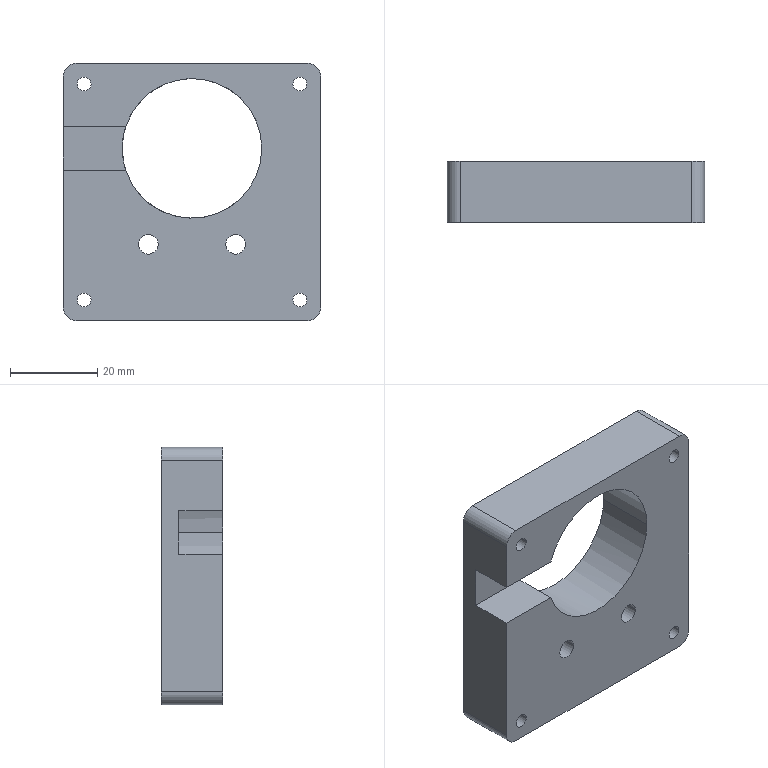Component | SolidWorks | MotorPlate-1 | 1 solid | 33 faces | box 59 x 14 x 59 mm | volume 34785 mm3 | cylinder 22 | plane 11 | commonest cylinder face diameters 3.2 x8 8 x4 4.5 x4 6 x4 32 x2 | material 6061 Alloy
STEP:
#1=CARTESIAN_POINT('',(-2.148,0.2347,12.047));
#2=VERTEX_POINT('',#1);
#3=CARTESIAN_POINT('',(-2.462,0.2347,12.047));
#4=VERTEX_POINT('',#3);
#5=CARTESIAN_POINT('',(-2.305,0.2347,12.047));
#6=DIRECTION('',(-0.,1.,-0.));
#7=DIRECTION('',(-1.,-0.,0.));
#8=AXIS2_PLACEMENT_3D('',#5,#6,#7);
#9=CIRCLE('',#8,0.1575);
#10=EDGE_CURVE('',#2,#4,#9,.T.);
#11=ORIENTED_EDGE('',*,*,#10,.F.);
#12=CARTESIAN_POINT('',(-2.148,0.4118,12.047));
#13=VERTEX_POINT('',#12);
#14=CARTESIAN_POINT('',(-2.148,0.2347,12.047));
#15=DIRECTION('',(-0.,1.,-0.));
#16=VECTOR('',#15,39.37);
#17=LINE('',#14,#16);
#18=EDGE_CURVE('',#2,#13,#17,.T.);
#19=ORIENTED_EDGE('',*,*,#18,.T.);
#20=CARTESIAN_POINT('',(-2.462,0.4118,12.047));
#21=VERTEX_POINT('',#20);
#22=CARTESIAN_POINT('',(-2.305,0.4118,12.047));
#23=DIRECTION('',(-0.,1.,-0.));
#24=DIRECTION('',(-1.,-0.,0.));
#25=AXIS2_PLACEMENT_3D('',#22,#23,#24);
#26=CIRCLE('',#25,0.1575);
#27=EDGE_CURVE('',#13,#21,#26,.T.);
#28=ORIENTED_EDGE('',*,*,#27,.T.);
#29=CARTESIAN_POINT('',(-2.462,0.2347,12.047));
#30=DIRECTION('',(-0.,1.,-0.));
#31=VECTOR('',#30,39.37);
#32=LINE('',#29,#31);
#33=EDGE_CURVE('',#4,#21,#32,.T.);
#34=ORIENTED_EDGE('',*,*,#33,.F.);
#35=EDGE_LOOP('',(#11,#19,#28,#34));
#36=FACE_OUTER_BOUND('',#35,.T.);
#37=CARTESIAN_POINT('',(-2.305,0.2347,12.047));
#38=DIRECTION('',(-0.,1.,-0.));
#39=DIRECTION('',(-1.,-0.,0.));
#40=AXIS2_PLACEMENT_3D('',#37,#38,#39);
#41=CYLINDRICAL_SURFACE('',#40,0.1575);
#42=ADVANCED_FACE('',(#36),#41,.F.);
#43=CARTESIAN_POINT('',(-1.36,0.2347,12.047));
#44=VERTEX_POINT('',#43);
#45=CARTESIAN_POINT('',(-1.675,0.2347,12.047));
#46=VERTEX_POINT('',#45);
#47=CARTESIAN_POINT('',(-1.518,0.2347,12.047));
#48=DIRECTION('',(-0.,1.,-0.));
#49=DIRECTION('',(-1.,-0.,0.));
#50=AXIS2_PLACEMENT_3D('',#47,#48,#49);
#51=CIRCLE('',#50,0.1575);
#52=EDGE_CURVE('',#44,#46,#51,.T.);
#53=ORIENTED_EDGE('',*,*,#52,.F.);
#54=CARTESIAN_POINT('',(-1.36,0.4118,12.047));
#55=VERTEX_POINT('',#54);
#56=CARTESIAN_POINT('',(-1.36,0.2347,12.047));
#57=DIRECTION('',(-0.,1.,-0.));
#58=VECTOR('',#57,39.37);
#59=LINE('',#56,#58);
#60=EDGE_CURVE('',#44,#55,#59,.T.);
#61=ORIENTED_EDGE('',*,*,#60,.T.);
#62=CARTESIAN_POINT('',(-1.675,0.4118,12.047));
#63=VERTEX_POINT('',#62);
#64=CARTESIAN_POINT('',(-1.518,0.4118,12.047));
#65=DIRECTION('',(-0.,1.,-0.));
#66=DIRECTION('',(-1.,-0.,0.));
#67=AXIS2_PLACEMENT_3D('',#64,#65,#66);
#68=CIRCLE('',#67,0.1575);
#69=EDGE_CURVE('',#55,#63,#68,.T.);
#70=ORIENTED_EDGE('',*,*,#69,.T.);
#71=CARTESIAN_POINT('',(-1.675,0.2347,12.047));
#72=DIRECTION('',(-0.,1.,-0.));
#73=VECTOR('',#72,39.37);
#74=LINE('',#71,#73);
#75=EDGE_CURVE('',#46,#63,#74,.T.);
#76=ORIENTED_EDGE('',*,*,#75,.F.);
#77=EDGE_LOOP('',(#53,#61,#70,#76));
#78=FACE_OUTER_BOUND('',#77,.T.);
#79=CARTESIAN_POINT('',(-1.518,0.2347,12.047));
#80=DIRECTION('',(-0.,1.,-0.));
#81=DIRECTION('',(-1.,-0.,0.));
#82=AXIS2_PLACEMENT_3D('',#79,#80,#81);
#83=CYLINDRICAL_SURFACE('',#82,0.1575);
#84=ADVANCED_FACE('',(#78),#83,.F.);
#85=CARTESIAN_POINT('',(-0.8739,0.4118,11.545));
#86=VERTEX_POINT('',#85);
#87=CARTESIAN_POINT('',(-0.9999,0.4118,11.545));
#88=VERTEX_POINT('',#87);
#89=CARTESIAN_POINT('',(-0.9369,0.4118,11.545));
#90=DIRECTION('',(-0.,1.,-0.));
#91=DIRECTION('',(-1.,0.,0.));
#92=AXIS2_PLACEMENT_3D('',#89,#90,#91);
#93=CIRCLE('',#92,0.06299);
#94=EDGE_CURVE('',#86,#88,#93,.T.);
#95=ORIENTED_EDGE('',*,*,#94,.T.);
#96=CARTESIAN_POINT('',(-0.9999,-0.1394,11.545));
#97=VERTEX_POINT('',#96);
#98=CARTESIAN_POINT('',(-0.9999,0.4118,11.545));
#99=DIRECTION('',(0.,-1.,0.));
#100=VECTOR('',#99,39.37);
#101=LINE('',#98,#100);
#102=EDGE_CURVE('',#88,#97,#101,.T.);
#103=ORIENTED_EDGE('',*,*,#102,.T.);
#104=CARTESIAN_POINT('',(-0.8739,-0.1394,11.545));
#105=VERTEX_POINT('',#104);
#106=CARTESIAN_POINT('',(-0.9369,-0.1394,11.545));
#107=DIRECTION('',(-0.,1.,-0.));
#108=DIRECTION('',(-1.,-0.,0.));
#109=AXIS2_PLACEMENT_3D('',#106,#107,#108);
#110=CIRCLE('',#109,0.06299);
#111=EDGE_CURVE('',#105,#97,#110,.T.);
#112=ORIENTED_EDGE('',*,*,#111,.F.);
#113=CARTESIAN_POINT('',(-0.8739,0.4118,11.545));
#114=DIRECTION('',(0.,-1.,0.));
#115=VECTOR('',#114,39.37);
#116=LINE('',#113,#115);
#117=EDGE_CURVE('',#86,#105,#116,.T.);
#118=ORIENTED_EDGE('',*,*,#117,.F.);
#119=EDGE_LOOP('',(#95,#103,#112,#118));
#120=FACE_OUTER_BOUND('',#119,.T.);
#121=CARTESIAN_POINT('',(-0.9369,0.4118,11.545));
#122=DIRECTION('',(0.,-1.,0.));
#123=DIRECTION('',(1.,0.,0.));
#124=AXIS2_PLACEMENT_3D('',#121,#122,#123);
#125=CYLINDRICAL_SURFACE('',#124,0.06299);
#126=ADVANCED_FACE('',(#120),#125,.F.);
#127=CARTESIAN_POINT('',(-2.823,0.4118,11.545));
#128=VERTEX_POINT('',#127);
#129=CARTESIAN_POINT('',(-2.949,0.4118,11.545));
#130=VERTEX_POINT('',#129);
#131=CARTESIAN_POINT('',(-2.886,0.4118,11.545));
#132=DIRECTION('',(-0.,1.,-0.));
#133=DIRECTION('',(-1.,0.,0.));
#134=AXIS2_PLACEMENT_3D('',#131,#132,#133);
#135=CIRCLE('',#134,0.06299);
#136=EDGE_CURVE('',#128,#130,#135,.T.);
#137=ORIENTED_EDGE('',*,*,#136,.T.);
#138=CARTESIAN_POINT('',(-2.949,-0.1394,11.545));
#139=VERTEX_POINT('',#138);
#140=CARTESIAN_POINT('',(-2.949,0.4118,11.545));
#141=DIRECTION('',(0.,-1.,0.));
#142=VECTOR('',#141,39.37);
#143=LINE('',#140,#142);
#144=EDGE_CURVE('',#130,#139,#143,.T.);
#145=ORIENTED_EDGE('',*,*,#144,.T.);
#146=CARTESIAN_POINT('',(-2.823,-0.1394,11.545));
#147=VERTEX_POINT('',#146);
#148=CARTESIAN_POINT('',(-2.886,-0.1394,11.545));
#149=DIRECTION('',(-0.,1.,-0.));
#150=DIRECTION('',(-1.,-0.,0.));
#151=AXIS2_PLACEMENT_3D('',#148,#149,#150);
#152=CIRCLE('',#151,0.06299);
#153=EDGE_CURVE('',#147,#139,#152,.T.);
#154=ORIENTED_EDGE('',*,*,#153,.F.);
#155=CARTESIAN_POINT('',(-2.823,0.4118,11.545));
#156=DIRECTION('',(0.,-1.,0.));
#157=VECTOR('',#156,39.37);
#158=LINE('',#155,#157);
#159=EDGE_CURVE('',#128,#147,#158,.T.);
#160=ORIENTED_EDGE('',*,*,#159,.F.);
#161=EDGE_LOOP('',(#137,#145,#154,#160));
#162=FACE_OUTER_BOUND('',#161,.T.);
#163=CARTESIAN_POINT('',(-2.886,0.4118,11.545));
#164=DIRECTION('',(0.,-1.,0.));
#165=DIRECTION('',(1.,0.,0.));
#166=AXIS2_PLACEMENT_3D('',#163,#164,#165);
#167=CYLINDRICAL_SURFACE('',#166,0.06299);
#168=ADVANCED_FACE('',(#162),#167,.F.);
#169=CARTESIAN_POINT('',(-2.823,0.4118,13.494));
#170=VERTEX_POINT('',#169);
#171=CARTESIAN_POINT('',(-2.949,0.4118,13.494));
#172=VERTEX_POINT('',#171);
#173=CARTESIAN_POINT('',(-2.886,0.4118,13.494));
#174=DIRECTION('',(-0.,1.,-0.));
#175=DIRECTION('',(-1.,0.,0.));
#176=AXIS2_PLACEMENT_3D('',#173,#174,#175);
#177=CIRCLE('',#176,0.06299);
#178=EDGE_CURVE('',#170,#172,#177,.T.);
#179=ORIENTED_EDGE('',*,*,#178,.T.);
#180=CARTESIAN_POINT('',(-2.949,-0.1394,13.494));
#181=VERTEX_POINT('',#180);
#182=CARTESIAN_POINT('',(-2.949,0.4118,13.494));
#183=DIRECTION('',(0.,-1.,0.));
#184=VECTOR('',#183,39.37);
#185=LINE('',#182,#184);
#186=EDGE_CURVE('',#172,#181,#185,.T.);
#187=ORIENTED_EDGE('',*,*,#186,.T.);
#188=CARTESIAN_POINT('',(-2.823,-0.1394,13.494));
#189=VERTEX_POINT('',#188);
#190=CARTESIAN_POINT('',(-2.886,-0.1394,13.494));
#191=DIRECTION('',(-0.,1.,-0.));
#192=DIRECTION('',(-1.,-0.,0.));
#193=AXIS2_PLACEMENT_3D('',#190,#191,#192);
#194=CIRCLE('',#193,0.06299);
#195=EDGE_CURVE('',#189,#181,#194,.T.);
#196=ORIENTED_EDGE('',*,*,#195,.F.);
#197=CARTESIAN_POINT('',(-2.823,0.4118,13.494));
#198=DIRECTION('',(0.,-1.,0.));
#199=VECTOR('',#198,39.37);
#200=LINE('',#197,#199);
#201=EDGE_CURVE('',#170,#189,#200,.T.);
#202=ORIENTED_EDGE('',*,*,#201,.F.);
#203=EDGE_LOOP('',(#179,#187,#196,#202));
#204=FACE_OUTER_BOUND('',#203,.T.);
#205=CARTESIAN_POINT('',(-2.886,0.4118,13.494));
#206=DIRECTION('',(0.,-1.,0.));
#207=DIRECTION('',(1.,0.,0.));
#208=AXIS2_PLACEMENT_3D('',#205,#206,#207);
#209=CYLINDRICAL_SURFACE('',#208,0.06299);
#210=ADVANCED_FACE('',(#204),#209,.F.);
#211=CARTESIAN_POINT('',(-0.8739,0.4118,13.494));
#212=VERTEX_POINT('',#211);
#213=CARTESIAN_POINT('',(-0.9999,0.4118,13.494));
#214=VERTEX_POINT('',#213);
#215=CARTESIAN_POINT('',(-0.9369,0.4118,13.494));
#216=DIRECTION('',(-0.,1.,-0.));
#217=DIRECTION('',(-1.,0.,0.));
#218=AXIS2_PLACEMENT_3D('',#215,#216,#217);
#219=CIRCLE('',#218,0.06299);
#220=EDGE_CURVE('',#212,#214,#219,.T.);
#221=ORIENTED_EDGE('',*,*,#220,.T.);
#222=CARTESIAN_POINT('',(-0.9999,-0.1394,13.494));
#223=VERTEX_POINT('',#222);
#224=CARTESIAN_POINT('',(-0.9999,0.4118,13.494));
#225=DIRECTION('',(0.,-1.,0.));
#226=VECTOR('',#225,39.37);
#227=LINE('',#224,#226);
#228=EDGE_CURVE('',#214,#223,#227,.T.);
#229=ORIENTED_EDGE('',*,*,#228,.T.);
#230=CARTESIAN_POINT('',(-0.8739,-0.1394,13.494));
#231=VERTEX_POINT('',#230);
#232=CARTESIAN_POINT('',(-0.9369,-0.1394,13.494));
#233=DIRECTION('',(-0.,1.,-0.));
#234=DIRECTION('',(-1.,-0.,0.));
#235=AXIS2_PLACEMENT_3D('',#232,#233,#234);
#236=CIRCLE('',#235,0.06299);
#237=EDGE_CURVE('',#231,#223,#236,.T.);
#238=ORIENTED_EDGE('',*,*,#237,.F.);
#239=CARTESIAN_POINT('',(-0.8739,0.4118,13.494));
#240=DIRECTION('',(0.,-1.,0.));
#241=VECTOR('',#240,39.37);
#242=LINE('',#239,#241);
#243=EDGE_CURVE('',#212,#231,#242,.T.);
#244=ORIENTED_EDGE('',*,*,#243,.F.);
#245=EDGE_LOOP('',(#221,#229,#238,#244));
#246=FACE_OUTER_BOUND('',#245,.T.);
#247=CARTESIAN_POINT('',(-0.9369,0.4118,13.494));
#248=DIRECTION('',(0.,-1.,0.));
#249=DIRECTION('',(1.,0.,0.));
#250=AXIS2_PLACEMENT_3D('',#247,#248,#249);
#251=CYLINDRICAL_SURFACE('',#250,0.06299);
#252=ADVANCED_FACE('',(#246),#251,.F.);
#253=CARTESIAN_POINT('',(-1.429,0.2347,12.047));
#254=VERTEX_POINT('',#253);
#255=CARTESIAN_POINT('',(-1.606,0.2347,12.047));
#256=VERTEX_POINT('',#255);
#257=CARTESIAN_POINT('',(-1.518,0.2347,12.047));
#258=DIRECTION('',(-0.,1.,-0.));
#259=DIRECTION('',(-1.,-0.,0.));
#260=AXIS2_PLACEMENT_3D('',#257,#258,#259);
#261=CIRCLE('',#260,0.08858);
#262=EDGE_CURVE('',#254,#256,#261,.T.);
#263=ORIENTED_EDGE('',*,*,#262,.T.);
#264=CARTESIAN_POINT('',(-1.606,-0.1394,12.047));
#265=VERTEX_POINT('',#264);
#266=CARTESIAN_POINT('',(-1.606,0.4118,12.047));
#267=DIRECTION('',(0.,-1.,0.));
#268=VECTOR('',#267,39.37);
#269=LINE('',#266,#268);
#270=EDGE_CURVE('',#256,#265,#269,.T.);
#271=ORIENTED_EDGE('',*,*,#270,.T.);
#272=CARTESIAN_POINT('',(-1.429,-0.1394,12.047));
#273=VERTEX_POINT('',#272);
#274=CARTESIAN_POINT('',(-1.518,-0.1394,12.047));
#275=DIRECTION('',(-0.,1.,-0.));
#276=DIRECTION('',(-1.,-0.,0.));
#277=AXIS2_PLACEMENT_3D('',#274,#275,#276);
#278=CIRCLE('',#277,0.08858);
#279=EDGE_CURVE('',#273,#265,#278,.T.);
#280=ORIENTED_EDGE('',*,*,#279,.F.);
#281=CARTESIAN_POINT('',(-1.429,0.4118,12.047));
#282=DIRECTION('',(0.,-1.,0.));
#283=VECTOR('',#282,39.37);
#284=LINE('',#281,#283);
#285=EDGE_CURVE('',#254,#273,#284,.T.);
#286=ORIENTED_EDGE('',*,*,#285,.F.);
#287=EDGE_LOOP('',(#263,#271,#280,#286));
#288=FACE_OUTER_BOUND('',#287,.T.);
#289=CARTESIAN_POINT('',(-1.518,0.4118,12.047));
#290=DIRECTION('',(0.,-1.,0.));
#291=DIRECTION('',(1.,0.,0.));
#292=AXIS2_PLACEMENT_3D('',#289,#290,#291);
#293=CYLINDRICAL_SURFACE('',#292,0.08858);
#294=ADVANCED_FACE('',(#288),#293,.F.);
#295=CARTESIAN_POINT('',(-2.216,0.2347,12.047));
#296=VERTEX_POINT('',#295);
#297=CARTESIAN_POINT('',(-2.394,0.2347,12.047));
#298=VERTEX_POINT('',#297);
#299=CARTESIAN_POINT('',(-2.305,0.2347,12.047));
#300=DIRECTION('',(-0.,1.,-0.));
#301=DIRECTION('',(-1.,-0.,0.));
#302=AXIS2_PLACEMENT_3D('',#299,#300,#301);
#303=CIRCLE('',#302,0.08858);
#304=EDGE_CURVE('',#296,#298,#303,.T.);
#305=ORIENTED_EDGE('',*,*,#304,.T.);
#306=CARTESIAN_POINT('',(-2.394,-0.1394,12.047));
#307=VERTEX_POINT('',#306);
#308=CARTESIAN_POINT('',(-2.394,0.4118,12.047));
#309=DIRECTION('',(0.,-1.,0.));
#310=VECTOR('',#309,39.37);
#311=LINE('',#308,#310);
#312=EDGE_CURVE('',#298,#307,#311,.T.);
#313=ORIENTED_EDGE('',*,*,#312,.T.);
#314=CARTESIAN_POINT('',(-2.216,-0.1394,12.047));
#315=VERTEX_POINT('',#314);
#316=CARTESIAN_POINT('',(-2.305,-0.1394,12.047));
#317=DIRECTION('',(-0.,1.,-0.));
#318=DIRECTION('',(-1.,-0.,0.));
#319=AXIS2_PLACEMENT_3D('',#316,#317,#318);
#320=CIRCLE('',#319,0.08858);
#321=EDGE_CURVE('',#315,#307,#320,.T.);
#322=ORIENTED_EDGE('',*,*,#321,.F.);
#323=CARTESIAN_POINT('',(-2.216,0.4118,12.047));
#324=DIRECTION('',(0.,-1.,0.));
#325=VECTOR('',#324,39.37);
#326=LINE('',#323,#325);
#327=EDGE_CURVE('',#296,#315,#326,.T.);
#328=ORIENTED_EDGE('',*,*,#327,.F.);
#329=EDGE_LOOP('',(#305,#313,#322,#328));
#330=FACE_OUTER_BOUND('',#329,.T.);
#331=CARTESIAN_POINT('',(-2.305,0.4118,12.047));
#332=DIRECTION('',(0.,-1.,0.));
#333=DIRECTION('',(1.,0.,0.));
#334=AXIS2_PLACEMENT_3D('',#331,#332,#333);
#335=CYLINDRICAL_SURFACE('',#334,0.08858);
#336=ADVANCED_FACE('',(#330),#335,.F.);
#337=CARTESIAN_POINT('',(-1.281,0.4118,12.913));
#338=VERTEX_POINT('',#337);
#339=CARTESIAN_POINT('',(-2.541,0.4118,12.913));
#340=VERTEX_POINT('',#339);
#341=CARTESIAN_POINT('',(-1.911,0.4118,12.913));
#342=DIRECTION('',(-0.,1.,-0.));
#343=DIRECTION('',(-1.,-0.,0.));
#344=AXIS2_PLACEMENT_3D('',#341,#342,#343);
#345=CIRCLE('',#344,0.6299);
#346=EDGE_CURVE('',#338,#340,#345,.T.);
#347=ORIENTED_EDGE('',*,*,#346,.T.);
#348=CARTESIAN_POINT('',(-2.541,0.2543,12.913));
#349=VERTEX_POINT('',#348);
#350=CARTESIAN_POINT('',(-2.541,0.4118,12.913));
#351=DIRECTION('',(0.,-1.,0.));
#352=VECTOR('',#351,39.37);
#353=LINE('',#350,#352);
#354=EDGE_CURVE('',#340,#349,#353,.T.);
#355=ORIENTED_EDGE('',*,*,#354,.T.);
#356=CARTESIAN_POINT('',(-2.51,0.2543,12.717));
#357=VERTEX_POINT('',#356);
#358=CARTESIAN_POINT('',(-1.911,0.2543,12.913));
#359=DIRECTION('',(0.,-1.,0.));
#360=DIRECTION('',(1.,0.,-0.));
#361=AXIS2_PLACEMENT_3D('',#358,#359,#360);
#362=CIRCLE('',#361,0.6299);
#363=EDGE_CURVE('',#349,#357,#362,.T.);
#364=ORIENTED_EDGE('',*,*,#363,.T.);
#365=CARTESIAN_POINT('',(-2.51,-0.1394,12.717));
#366=VERTEX_POINT('',#365);
#367=CARTESIAN_POINT('',(-2.51,0.4118,12.717));
#368=DIRECTION('',(0.,-1.,0.));
#369=VECTOR('',#368,39.37);
#370=LINE('',#367,#369);
#371=EDGE_CURVE('',#357,#366,#370,.T.);
#372=ORIENTED_EDGE('',*,*,#371,.T.);
#373=CARTESIAN_POINT('',(-1.281,-0.1394,12.913));
#374=VERTEX_POINT('',#373);
#375=CARTESIAN_POINT('',(-1.911,-0.1394,12.913));
#376=DIRECTION('',(-0.,1.,-0.));
#377=DIRECTION('',(-1.,-0.,0.));
#378=AXIS2_PLACEMENT_3D('',#375,#376,#377);
#379=CIRCLE('',#378,0.6299);
#380=EDGE_CURVE('',#374,#366,#379,.T.);
#381=ORIENTED_EDGE('',*,*,#380,.F.);
#382=CARTESIAN_POINT('',(-1.281,0.4118,12.913));
#383=DIRECTION('',(0.,-1.,0.));
#384=VECTOR('',#383,39.37);
#385=LINE('',#382,#384);
#386=EDGE_CURVE('',#338,#374,#385,.T.);
#387=ORIENTED_EDGE('',*,*,#386,.F.);
#388=EDGE_LOOP('',(#347,#355,#364,#372,#381,#387));
#389=FACE_OUTER_BOUND('',#388,.T.);
#390=CARTESIAN_POINT('',(-1.911,0.4118,12.913));
#391=DIRECTION('',(0.,-1.,0.));
#392=DIRECTION('',(1.,0.,-0.));
#393=AXIS2_PLACEMENT_3D('',#390,#391,#392);
#394=CYLINDRICAL_SURFACE('',#393,0.6299);
#395=ADVANCED_FACE('',(#389),#394,.F.);
#396=ORIENTED_EDGE('',*,*,#321,.T.);
#397=CARTESIAN_POINT('',(-2.305,-0.1394,12.047));
#398=DIRECTION('',(-0.,1.,-0.));
#399=DIRECTION('',(-1.,-0.,0.));
#400=AXIS2_PLACEMENT_3D('',#397,#398,#399);
#401=CIRCLE('',#400,0.08858);
#402=EDGE_CURVE('',#307,#315,#401,.T.);
#403=ORIENTED_EDGE('',*,*,#402,.T.);
#404=EDGE_LOOP('',(#396,#403));
#405=FACE_BOUND('',#404,.T.);
#406=ORIENTED_EDGE('',*,*,#279,.T.);
#407=CARTESIAN_POINT('',(-1.518,-0.1394,12.047));
#408=DIRECTION('',(-0.,1.,-0.));
#409=DIRECTION('',(-1.,-0.,0.));
#410=AXIS2_PLACEMENT_3D('',#407,#408,#409);
#411=CIRCLE('',#410,0.08858);
#412=EDGE_CURVE('',#265,#273,#411,.T.);
#413=ORIENTED_EDGE('',*,*,#412,.T.);
#414=EDGE_LOOP('',(#406,#413));
#415=FACE_BOUND('',#414,.T.);
#416=ORIENTED_EDGE('',*,*,#111,.T.);
#417=CARTESIAN_POINT('',(-0.9369,-0.1394,11.545));
#418=DIRECTION('',(-0.,1.,-0.));
#419=DIRECTION('',(-1.,-0.,0.));
#420=AXIS2_PLACEMENT_3D('',#417,#418,#419);
#421=CIRCLE('',#420,0.06299);
#422=EDGE_CURVE('',#97,#105,#421,.T.);
#423=ORIENTED_EDGE('',*,*,#422,.T.);
#424=EDGE_LOOP('',(#416,#423));
#425=FACE_BOUND('',#424,.T.);
#426=ORIENTED_EDGE('',*,*,#153,.T.);
#427=CARTESIAN_POINT('',(-2.886,-0.1394,11.545));
#428=DIRECTION('',(-0.,1.,-0.));
#429=DIRECTION('',(-1.,-0.,0.));
#430=AXIS2_PLACEMENT_3D('',#427,#428,#429);
#431=CIRCLE('',#430,0.06299);
#432=EDGE_CURVE('',#139,#147,#431,.T.);
#433=ORIENTED_EDGE('',*,*,#432,.T.);
#434=EDGE_LOOP('',(#426,#433));
#435=FACE_BOUND('',#434,.T.);
#436=ORIENTED_EDGE('',*,*,#195,.T.);
#437=CARTESIAN_POINT('',(-2.886,-0.1394,13.494));
#438=DIRECTION('',(-0.,1.,-0.));
#439=DIRECTION('',(-1.,-0.,0.));
#440=AXIS2_PLACEMENT_3D('',#437,#438,#439);
#441=CIRCLE('',#440,0.06299);
#442=EDGE_CURVE('',#181,#189,#441,.T.);
#443=ORIENTED_EDGE('',*,*,#442,.T.);
#444=EDGE_LOOP('',(#436,#443));
#445=FACE_BOUND('',#444,.T.);
#446=ORIENTED_EDGE('',*,*,#237,.T.);
#447=CARTESIAN_POINT('',(-0.9369,-0.1394,13.494));
#448=DIRECTION('',(-0.,1.,-0.));
#449=DIRECTION('',(-1.,-0.,0.));
#450=AXIS2_PLACEMENT_3D('',#447,#448,#449);
#451=CIRCLE('',#450,0.06299);
#452=EDGE_CURVE('',#223,#231,#451,.T.);
#453=ORIENTED_EDGE('',*,*,#452,.T.);
#454=EDGE_LOOP('',(#446,#453));
#455=FACE_BOUND('',#454,.T.);
#456=CARTESIAN_POINT('',(-2.955,-0.1394,13.681));
#457=VERTEX_POINT('',#456);
#458=CARTESIAN_POINT('',(-0.868,-0.1394,13.681));
#459=VERTEX_POINT('',#458);
#460=CARTESIAN_POINT('',(-0.7499,-0.1394,13.681));
#461=DIRECTION('',(1.,0.,-0.));
#462=VECTOR('',#461,39.37);
#463=LINE('',#460,#462);
#464=EDGE_CURVE('',#457,#459,#463,.T.);
#465=ORIENTED_EDGE('',*,*,#464,.F.);
#466=CARTESIAN_POINT('',(-3.073,-0.1394,13.563));
#467=VERTEX_POINT('',#466);
#468=CARTESIAN_POINT('',(-2.955,-0.1394,13.563));
#469=DIRECTION('',(0.,-1.,0.));
#470=DIRECTION('',(-1.,-0.,0.));
#471=AXIS2_PLACEMENT_3D('',#468,#469,#470);
#472=CIRCLE('',#471,0.1181);
#473=EDGE_CURVE('',#457,#467,#472,.T.);
#474=ORIENTED_EDGE('',*,*,#473,.T.);
#475=CARTESIAN_POINT('',(-3.073,-0.1394,13.11));
#476=VERTEX_POINT('',#475);
#477=CARTESIAN_POINT('',(-3.073,-0.1394,13.681));
#478=DIRECTION('',(0.,0.,1.));
#479=VECTOR('',#478,39.37);
#480=LINE('',#477,#479);
#481=EDGE_CURVE('',#476,#467,#480,.T.);
#482=ORIENTED_EDGE('',*,*,#481,.F.);
#483=CARTESIAN_POINT('',(-2.51,-0.1394,13.11));
#484=VERTEX_POINT('',#483);
#485=CARTESIAN_POINT('',(-3.073,-0.1394,13.11));
#486=DIRECTION('',(1.,0.,-0.));
#487=VECTOR('',#486,39.37);
#488=LINE('',#485,#487);
#489=EDGE_CURVE('',#476,#484,#488,.T.);
#490=ORIENTED_EDGE('',*,*,#489,.T.);
#491=CARTESIAN_POINT('',(-1.911,-0.1394,12.913));
#492=DIRECTION('',(-0.,1.,-0.));
#493=DIRECTION('',(-1.,-0.,0.));
#494=AXIS2_PLACEMENT_3D('',#491,#492,#493);
#495=CIRCLE('',#494,0.6299);
#496=EDGE_CURVE('',#484,#374,#495,.T.);
#497=ORIENTED_EDGE('',*,*,#496,.T.);
#498=ORIENTED_EDGE('',*,*,#380,.T.);
#499=CARTESIAN_POINT('',(-3.073,-0.1394,12.717));
#500=VERTEX_POINT('',#499);
#501=CARTESIAN_POINT('',(-3.073,-0.1394,12.717));
#502=DIRECTION('',(-1.,-0.,0.));
#503=VECTOR('',#502,39.37);
#504=LINE('',#501,#503);
#505=EDGE_CURVE('',#366,#500,#504,.T.);
#506=ORIENTED_EDGE('',*,*,#505,.T.);
#507=CARTESIAN_POINT('',(-3.073,-0.1394,11.476));
#508=VERTEX_POINT('',#507);
#509=CARTESIAN_POINT('',(-3.073,-0.1394,13.681));
#510=DIRECTION('',(0.,0.,1.));
#511=VECTOR('',#510,39.37);
#512=LINE('',#509,#511);
#513=EDGE_CURVE('',#508,#500,#512,.T.);
#514=ORIENTED_EDGE('',*,*,#513,.F.);
#515=CARTESIAN_POINT('',(-2.955,-0.1394,11.358));
#516=VERTEX_POINT('',#515);
#517=CARTESIAN_POINT('',(-2.955,-0.1394,11.476));
#518=DIRECTION('',(0.,-1.,0.));
#519=DIRECTION('',(-1.,-0.,0.));
#520=AXIS2_PLACEMENT_3D('',#517,#518,#519);
#521=CIRCLE('',#520,0.1181);
#522=EDGE_CURVE('',#508,#516,#521,.T.);
#523=ORIENTED_EDGE('',*,*,#522,.T.);
#524=CARTESIAN_POINT('',(-0.868,-0.1394,11.358));
#525=VERTEX_POINT('',#524);
#526=CARTESIAN_POINT('',(-0.7499,-0.1394,11.358));
#527=DIRECTION('',(-1.,-0.,0.));
#528=VECTOR('',#527,39.37);
#529=LINE('',#526,#528);
#530=EDGE_CURVE('',#525,#516,#529,.T.);
#531=ORIENTED_EDGE('',*,*,#530,.F.);
#532=CARTESIAN_POINT('',(-0.7499,-0.1394,11.476));
#533=VERTEX_POINT('',#532);
#534=CARTESIAN_POINT('',(-0.868,-0.1394,11.476));
#535=DIRECTION('',(0.,-1.,0.));
#536=DIRECTION('',(-1.,-0.,0.));
#537=AXIS2_PLACEMENT_3D('',#534,#535,#536);
#538=CIRCLE('',#537,0.1181);
#539=EDGE_CURVE('',#525,#533,#538,.T.);
#540=ORIENTED_EDGE('',*,*,#539,.T.);
#541=CARTESIAN_POINT('',(-0.7499,-0.1394,13.563));
#542=VERTEX_POINT('',#541);
#543=CARTESIAN_POINT('',(-0.7499,-0.1394,13.681));
#544=DIRECTION('',(-0.,-0.,-1.));
#545=VECTOR('',#544,39.37);
#546=LINE('',#543,#545);
#547=EDGE_CURVE('',#542,#533,#546,.T.);
#548=ORIENTED_EDGE('',*,*,#547,.F.);
#549=CARTESIAN_POINT('',(-0.868,-0.1394,13.563));
#550=DIRECTION('',(0.,-1.,0.));
#551=DIRECTION('',(-1.,-0.,0.));
#552=AXIS2_PLACEMENT_3D('',#549,#550,#551);
#553=CIRCLE('',#552,0.1181);
#554=EDGE_CURVE('',#542,#459,#553,.T.);
#555=ORIENTED_EDGE('',*,*,#554,.T.);
#556=EDGE_LOOP('',(#465,#474,#482,#490,#497,#498,#506,#514,#523,#531,#540,#548,#555));
#557=FACE_OUTER_BOUND('',#556,.T.);
#558=CARTESIAN_POINT('',(-0.7499,-0.1394,11.358));
#559=DIRECTION('',(-0.,1.,-0.));
#560=DIRECTION('',(-1.,-0.,0.));
#561=AXIS2_PLACEMENT_3D('',#558,#559,#560);
#562=PLANE('',#561);
#563=ADVANCED_FACE('',(#405,#415,#425,#435,#445,#455,#557),#562,.F.);
#564=ORIENTED_EDGE('',*,*,#481,.T.);
#565=CARTESIAN_POINT('',(-3.073,0.4118,13.563));
#566=VERTEX_POINT('',#565);
#567=CARTESIAN_POINT('',(-3.073,0.4118,13.563));
#568=DIRECTION('',(-0.,1.,-0.));
#569=VECTOR('',#568,39.37);
#570=LINE('',#567,#569);
#571=EDGE_CURVE('',#467,#566,#570,.T.);
#572=ORIENTED_EDGE('',*,*,#571,.T.);
#573=CARTESIAN_POINT('',(-3.073,0.4118,11.476));
#574=VERTEX_POINT('',#573);
#575=CARTESIAN_POINT('',(-3.073,0.4118,13.681));
#576=DIRECTION('',(0.,0.,1.));
#577=VECTOR('',#576,39.37);
#578=LINE('',#575,#577);
#579=EDGE_CURVE('',#574,#566,#578,.T.);
#580=ORIENTED_EDGE('',*,*,#579,.F.);
#581=CARTESIAN_POINT('',(-3.073,0.4118,11.476));
#582=DIRECTION('',(0.,-1.,0.));
#583=VECTOR('',#582,39.37);
#584=LINE('',#581,#583);
#585=EDGE_CURVE('',#574,#508,#584,.T.);
#586=ORIENTED_EDGE('',*,*,#585,.T.);
#587=ORIENTED_EDGE('',*,*,#513,.T.);
#588=CARTESIAN_POINT('',(-3.073,0.2543,12.717));
#589=VERTEX_POINT('',#588);
#590=CARTESIAN_POINT('',(-3.073,0.2543,12.717));
#591=DIRECTION('',(0.,-1.,0.));
#592=VECTOR('',#591,39.37);
#593=LINE('',#590,#592);
#594=EDGE_CURVE('',#589,#500,#593,.T.);
#595=ORIENTED_EDGE('',*,*,#594,.F.);
#596=CARTESIAN_POINT('',(-3.073,0.2543,13.11));
#597=VERTEX_POINT('',#596);
#598=CARTESIAN_POINT('',(-3.073,0.2543,13.11));
#599=DIRECTION('',(0.,0.,1.));
#600=VECTOR('',#599,39.37);
#601=LINE('',#598,#600);
#602=EDGE_CURVE('',#589,#597,#601,.T.);
#603=ORIENTED_EDGE('',*,*,#602,.T.);
#604=CARTESIAN_POINT('',(-3.073,0.2543,13.11));
#605=DIRECTION('',(0.,-1.,0.));
#606=VECTOR('',#605,39.37);
#607=LINE('',#604,#606);
#608=EDGE_CURVE('',#597,#476,#607,.T.);
#609=ORIENTED_EDGE('',*,*,#608,.T.);
#610=EDGE_LOOP('',(#564,#572,#580,#586,#587,#595,#603,#609));
#611=FACE_OUTER_BOUND('',#610,.T.);
#612=CARTESIAN_POINT('',(-3.073,0.4118,13.681));
#613=DIRECTION('',(1.,0.,-0.));
#614=DIRECTION('',(-0.,1.,-0.));
#615=AXIS2_PLACEMENT_3D('',#612,#613,#614);
#616=PLANE('',#615);
#617=ADVANCED_FACE('',(#611),#616,.F.);
#618=ORIENTED_EDGE('',*,*,#354,.F.);
#619=CARTESIAN_POINT('',(-1.911,0.4118,12.913));
#620=DIRECTION('',(-0.,1.,-0.));
#621=DIRECTION('',(-1.,-0.,0.));
#622=AXIS2_PLACEMENT_3D('',#619,#620,#621);
#623=CIRCLE('',#622,0.6299);
#624=EDGE_CURVE('',#340,#338,#623,.T.);
#625=ORIENTED_EDGE('',*,*,#624,.T.);
#626=ORIENTED_EDGE('',*,*,#386,.T.);
#627=ORIENTED_EDGE('',*,*,#496,.F.);
#628=CARTESIAN_POINT('',(-2.51,0.2543,13.11));
#629=VERTEX_POINT('',#628);
#630=CARTESIAN_POINT('',(-2.51,0.4118,13.11));
#631=DIRECTION('',(-0.,1.,-0.));
#632=VECTOR('',#631,39.37);
#633=LINE('',#630,#632);
#634=EDGE_CURVE('',#484,#629,#633,.T.);
#635=ORIENTED_EDGE('',*,*,#634,.T.);
#636=CARTESIAN_POINT('',(-1.911,0.2543,12.913));
#637=DIRECTION('',(0.,-1.,0.));
#638=DIRECTION('',(1.,0.,-0.));
#639=AXIS2_PLACEMENT_3D('',#636,#637,#638);
#640=CIRCLE('',#639,0.6299);
#641=EDGE_CURVE('',#629,#349,#640,.T.);
#642=ORIENTED_EDGE('',*,*,#641,.T.);
#643=EDGE_LOOP('',(#618,#625,#626,#627,#635,#642));
#644=FACE_OUTER_BOUND('',#643,.T.);
#645=CARTESIAN_POINT('',(-1.911,0.4118,12.913));
#646=DIRECTION('',(0.,-1.,0.));
#647=DIRECTION('',(1.,0.,-0.));
#648=AXIS2_PLACEMENT_3D('',#645,#646,#647);
#649=CYLINDRICAL_SURFACE('',#648,0.6299);
#650=ADVANCED_FACE('',(#644),#649,.F.);
#651=ORIENTED_EDGE('',*,*,#312,.F.);
#652=CARTESIAN_POINT('',(-2.305,0.2347,12.047));
#653=DIRECTION('',(-0.,1.,-0.));
#654=DIRECTION('',(-1.,-0.,0.));
#655=AXIS2_PLACEMENT_3D('',#652,#653,#654);
#656=CIRCLE('',#655,0.08858);
#657=EDGE_CURVE('',#298,#296,#656,.T.);
#658=ORIENTED_EDGE('',*,*,#657,.T.);
#659=ORIENTED_EDGE('',*,*,#327,.T.);
#660=ORIENTED_EDGE('',*,*,#402,.F.);
#661=EDGE_LOOP('',(#651,#658,#659,#660));
#662=FACE_OUTER_BOUND('',#661,.T.);
#663=CARTESIAN_POINT('',(-2.305,0.4118,12.047));
#664=DIRECTION('',(0.,-1.,0.));
#665=DIRECTION('',(1.,0.,0.));
#666=AXIS2_PLACEMENT_3D('',#663,#664,#665);
#667=CYLINDRICAL_SURFACE('',#666,0.08858);
#668=ADVANCED_FACE('',(#662),#667,.F.);
#669=ORIENTED_EDGE('',*,*,#270,.F.);
#670=CARTESIAN_POINT('',(-1.518,0.2347,12.047));
#671=DIRECTION('',(-0.,1.,-0.));
#672=DIRECTION('',(-1.,-0.,0.));
#673=AXIS2_PLACEMENT_3D('',#670,#671,#672);
#674=CIRCLE('',#673,0.08858);
#675=EDGE_CURVE('',#256,#254,#674,.T.);
#676=ORIENTED_EDGE('',*,*,#675,.T.);
#677=ORIENTED_EDGE('',*,*,#285,.T.);
#678=ORIENTED_EDGE('',*,*,#412,.F.);
#679=EDGE_LOOP('',(#669,#676,#677,#678));
#680=FACE_OUTER_BOUND('',#679,.T.);
#681=CARTESIAN_POINT('',(-1.518,0.4118,12.047));
#682=DIRECTION('',(0.,-1.,0.));
#683=DIRECTION('',(1.,0.,0.));
#684=AXIS2_PLACEMENT_3D('',#681,#682,#683);
#685=CYLINDRICAL_SURFACE('',#684,0.08858);
#686=ADVANCED_FACE('',(#680),#685,.F.);
#687=CARTESIAN_POINT('',(-2.305,0.4118,12.047));
#688=DIRECTION('',(-0.,1.,-0.));
#689=DIRECTION('',(-1.,-0.,0.));
#690=AXIS2_PLACEMENT_3D('',#687,#688,#689);
#691=CIRCLE('',#690,0.1575);
#692=EDGE_CURVE('',#21,#13,#691,.T.);
#693=ORIENTED_EDGE('',*,*,#692,.F.);
#694=ORIENTED_EDGE('',*,*,#27,.F.);
#695=EDGE_LOOP('',(#693,#694));
#696=FACE_BOUND('',#695,.T.);
#697=CARTESIAN_POINT('',(-1.518,0.4118,12.047));
#698=DIRECTION('',(-0.,1.,-0.));
#699=DIRECTION('',(-1.,-0.,0.));
#700=AXIS2_PLACEMENT_3D('',#697,#698,#699);
#701=CIRCLE('',#700,0.1575);
#702=EDGE_CURVE('',#63,#55,#701,.T.);
#703=ORIENTED_EDGE('',*,*,#702,.F.);
#704=ORIENTED_EDGE('',*,*,#69,.F.);
#705=EDGE_LOOP('',(#703,#704));
#706=FACE_BOUND('',#705,.T.);
#707=ORIENTED_EDGE('',*,*,#94,.F.);
#708=CARTESIAN_POINT('',(-0.9369,0.4118,11.545));
#709=DIRECTION('',(-0.,1.,-0.));
#710=DIRECTION('',(-1.,0.,0.));
#711=AXIS2_PLACEMENT_3D('',#708,#709,#710);
#712=CIRCLE('',#711,0.06299);
#713=EDGE_CURVE('',#88,#86,#712,.T.);
#714=ORIENTED_EDGE('',*,*,#713,.F.);
#715=EDGE_LOOP('',(#707,#714));
#716=FACE_BOUND('',#715,.T.);
#717=ORIENTED_EDGE('',*,*,#178,.F.);
#718=CARTESIAN_POINT('',(-2.886,0.4118,13.494));
#719=DIRECTION('',(-0.,1.,-0.));
#720=DIRECTION('',(-1.,0.,0.));
#721=AXIS2_PLACEMENT_3D('',#718,#719,#720);
#722=CIRCLE('',#721,0.06299);
#723=EDGE_CURVE('',#172,#170,#722,.T.);
#724=ORIENTED_EDGE('',*,*,#723,.F.);
#725=EDGE_LOOP('',(#717,#724));
#726=FACE_BOUND('',#725,.T.);
#727=ORIENTED_EDGE('',*,*,#579,.T.);
#728=CARTESIAN_POINT('',(-2.955,0.4118,13.681));
#729=VERTEX_POINT('',#728);
#730=CARTESIAN_POINT('',(-2.955,0.4118,13.563));
#731=DIRECTION('',(-0.,1.,-0.));
#732=DIRECTION('',(-1.,-0.,0.));
#733=AXIS2_PLACEMENT_3D('',#730,#731,#732);
#734=CIRCLE('',#733,0.1181);
#735=EDGE_CURVE('',#566,#729,#734,.T.);
#736=ORIENTED_EDGE('',*,*,#735,.T.);
#737=CARTESIAN_POINT('',(-0.868,0.4118,13.681));
#738=VERTEX_POINT('',#737);
#739=CARTESIAN_POINT('',(-0.7499,0.4118,13.681));
#740=DIRECTION('',(1.,0.,-0.));
#741=VECTOR('',#740,39.37);
#742=LINE('',#739,#741);
#743=EDGE_CURVE('',#729,#738,#742,.T.);
#744=ORIENTED_EDGE('',*,*,#743,.T.);
#745=CARTESIAN_POINT('',(-0.7499,0.4118,13.563));
#746=VERTEX_POINT('',#745);
#747=CARTESIAN_POINT('',(-0.868,0.4118,13.563));
#748=DIRECTION('',(-0.,1.,-0.));
#749=DIRECTION('',(-1.,-0.,0.));
#750=AXIS2_PLACEMENT_3D('',#747,#748,#749);
#751=CIRCLE('',#750,0.1181);
#752=EDGE_CURVE('',#738,#746,#751,.T.);
#753=ORIENTED_EDGE('',*,*,#752,.T.);
#754=CARTESIAN_POINT('',(-0.7499,0.4118,11.476));
#755=VERTEX_POINT('',#754);
#756=CARTESIAN_POINT('',(-0.7499,0.4118,13.681));
#757=DIRECTION('',(-0.,-0.,-1.));
#758=VECTOR('',#757,39.37);
#759=LINE('',#756,#758);
#760=EDGE_CURVE('',#746,#755,#759,.T.);
#761=ORIENTED_EDGE('',*,*,#760,.T.);
#762=CARTESIAN_POINT('',(-0.868,0.4118,11.358));
#763=VERTEX_POINT('',#762);
#764=CARTESIAN_POINT('',(-0.868,0.4118,11.476));
#765=DIRECTION('',(-0.,1.,-0.));
#766=DIRECTION('',(-1.,-0.,0.));
#767=AXIS2_PLACEMENT_3D('',#764,#765,#766);
#768=CIRCLE('',#767,0.1181);
#769=EDGE_CURVE('',#755,#763,#768,.T.);
#770=ORIENTED_EDGE('',*,*,#769,.T.);
#771=CARTESIAN_POINT('',(-2.955,0.4118,11.358));
#772=VERTEX_POINT('',#771);
#773=CARTESIAN_POINT('',(-0.7499,0.4118,11.358));
#774=DIRECTION('',(-1.,-0.,0.));
#775=VECTOR('',#774,39.37);
#776=LINE('',#773,#775);
#777=EDGE_CURVE('',#763,#772,#776,.T.);
#778=ORIENTED_EDGE('',*,*,#777,.T.);
#779=CARTESIAN_POINT('',(-2.955,0.4118,11.476));
#780=DIRECTION('',(-0.,1.,-0.));
#781=DIRECTION('',(-1.,-0.,0.));
#782=AXIS2_PLACEMENT_3D('',#779,#780,#781);
#783=CIRCLE('',#782,0.1181);
#784=EDGE_CURVE('',#772,#574,#783,.T.);
#785=ORIENTED_EDGE('',*,*,#784,.T.);
#786=EDGE_LOOP('',(#727,#736,#744,#753,#761,#770,#778,#785));
#787=FACE_OUTER_BOUND('',#786,.T.);
#788=ORIENTED_EDGE('',*,*,#220,.F.);
#789=CARTESIAN_POINT('',(-0.9369,0.4118,13.494));
#790=DIRECTION('',(-0.,1.,-0.));
#791=DIRECTION('',(-1.,0.,0.));
#792=AXIS2_PLACEMENT_3D('',#789,#790,#791);
#793=CIRCLE('',#792,0.06299);
#794=EDGE_CURVE('',#214,#212,#793,.T.);
#795=ORIENTED_EDGE('',*,*,#794,.F.);
#796=EDGE_LOOP('',(#788,#795));
#797=FACE_BOUND('',#796,.T.);
#798=ORIENTED_EDGE('',*,*,#136,.F.);
#799=CARTESIAN_POINT('',(-2.886,0.4118,11.545));
#800=DIRECTION('',(-0.,1.,-0.));
#801=DIRECTION('',(-1.,0.,0.));
#802=AXIS2_PLACEMENT_3D('',#799,#800,#801);
#803=CIRCLE('',#802,0.06299);
#804=EDGE_CURVE('',#130,#128,#803,.T.);
#805=ORIENTED_EDGE('',*,*,#804,.F.);
#806=EDGE_LOOP('',(#798,#805));
#807=FACE_BOUND('',#806,.T.);
#808=ORIENTED_EDGE('',*,*,#346,.F.);
#809=ORIENTED_EDGE('',*,*,#624,.F.);
#810=EDGE_LOOP('',(#808,#809));
#811=FACE_BOUND('',#810,.T.);
#812=CARTESIAN_POINT('',(-0.7499,0.4118,11.358));
#813=DIRECTION('',(-0.,1.,-0.));
#814=DIRECTION('',(-1.,-0.,0.));
#815=AXIS2_PLACEMENT_3D('',#812,#813,#814);
#816=PLANE('',#815);
#817=ADVANCED_FACE('',(#696,#706,#716,#726,#787,#797,#807,#811),#816,.T.);
#818=ORIENTED_EDGE('',*,*,#547,.T.);
#819=CARTESIAN_POINT('',(-0.7499,0.4118,11.476));
#820=DIRECTION('',(-0.,1.,-0.));
#821=VECTOR('',#820,39.37);
#822=LINE('',#819,#821);
#823=EDGE_CURVE('',#533,#755,#822,.T.);
#824=ORIENTED_EDGE('',*,*,#823,.T.);
#825=ORIENTED_EDGE('',*,*,#760,.F.);
#826=CARTESIAN_POINT('',(-0.7499,0.4118,13.563));
#827=DIRECTION('',(0.,-1.,0.));
#828=VECTOR('',#827,39.37);
#829=LINE('',#826,#828);
#830=EDGE_CURVE('',#746,#542,#829,.T.);
#831=ORIENTED_EDGE('',*,*,#830,.T.);
#832=EDGE_LOOP('',(#818,#824,#825,#831));
#833=FACE_OUTER_BOUND('',#832,.T.);
#834=CARTESIAN_POINT('',(-0.7499,0.4118,13.681));
#835=DIRECTION('',(-1.,-0.,0.));
#836=DIRECTION('',(0.,-1.,0.));
#837=AXIS2_PLACEMENT_3D('',#834,#835,#836);
#838=PLANE('',#837);
#839=ADVANCED_FACE('',(#833),#838,.F.);
#840=ORIENTED_EDGE('',*,*,#530,.T.);
#841=CARTESIAN_POINT('',(-2.955,0.4118,11.358));
#842=DIRECTION('',(-0.,1.,-0.));
#843=VECTOR('',#842,39.37);
#844=LINE('',#841,#843);
#845=EDGE_CURVE('',#516,#772,#844,.T.);
#846=ORIENTED_EDGE('',*,*,#845,.T.);
#847=ORIENTED_EDGE('',*,*,#777,.F.);
#848=CARTESIAN_POINT('',(-0.868,0.4118,11.358));
#849=DIRECTION('',(0.,-1.,0.));
#850=VECTOR('',#849,39.37);
#851=LINE('',#848,#850);
#852=EDGE_CURVE('',#763,#525,#851,.T.);
#853=ORIENTED_EDGE('',*,*,#852,.T.);
#854=EDGE_LOOP('',(#840,#846,#847,#853));
#855=FACE_OUTER_BOUND('',#854,.T.);
#856=CARTESIAN_POINT('',(-0.7499,0.4118,11.358));
#857=DIRECTION('',(0.,0.,1.));
#858=DIRECTION('',(-0.,1.,-0.));
#859=AXIS2_PLACEMENT_3D('',#856,#857,#858);
#860=PLANE('',#859);
#861=ADVANCED_FACE('',(#855),#860,.F.);
#862=ORIENTED_EDGE('',*,*,#743,.F.);
#863=CARTESIAN_POINT('',(-2.955,0.4118,13.681));
#864=DIRECTION('',(0.,-1.,0.));
#865=VECTOR('',#864,39.37);
#866=LINE('',#863,#865);
#867=EDGE_CURVE('',#729,#457,#866,.T.);
#868=ORIENTED_EDGE('',*,*,#867,.T.);
#869=ORIENTED_EDGE('',*,*,#464,.T.);
#870=CARTESIAN_POINT('',(-0.868,0.4118,13.681));
#871=DIRECTION('',(-0.,1.,-0.));
#872=VECTOR('',#871,39.37);
#873=LINE('',#870,#872);
#874=EDGE_CURVE('',#459,#738,#873,.T.);
#875=ORIENTED_EDGE('',*,*,#874,.T.);
#876=EDGE_LOOP('',(#862,#868,#869,#875));
#877=FACE_OUTER_BOUND('',#876,.T.);
#878=CARTESIAN_POINT('',(-0.7499,0.4118,13.681));
#879=DIRECTION('',(-0.,-0.,-1.));
#880=DIRECTION('',(0.,-1.,0.));
#881=AXIS2_PLACEMENT_3D('',#878,#879,#880);
#882=PLANE('',#881);
#883=ADVANCED_FACE('',(#877),#882,.F.);
#884=ORIENTED_EDGE('',*,*,#228,.F.);
#885=ORIENTED_EDGE('',*,*,#794,.T.);
#886=ORIENTED_EDGE('',*,*,#243,.T.);
#887=ORIENTED_EDGE('',*,*,#452,.F.);
#888=EDGE_LOOP('',(#884,#885,#886,#887));
#889=FACE_OUTER_BOUND('',#888,.T.);
#890=CARTESIAN_POINT('',(-0.9369,0.4118,13.494));
#891=DIRECTION('',(0.,-1.,0.));
#892=DIRECTION('',(1.,0.,0.));
#893=AXIS2_PLACEMENT_3D('',#890,#891,#892);
#894=CYLINDRICAL_SURFACE('',#893,0.06299);
#895=ADVANCED_FACE('',(#889),#894,.F.);
#896=ORIENTED_EDGE('',*,*,#186,.F.);
#897=ORIENTED_EDGE('',*,*,#723,.T.);
#898=ORIENTED_EDGE('',*,*,#201,.T.);
#899=ORIENTED_EDGE('',*,*,#442,.F.);
#900=EDGE_LOOP('',(#896,#897,#898,#899));
#901=FACE_OUTER_BOUND('',#900,.T.);
#902=CARTESIAN_POINT('',(-2.886,0.4118,13.494));
#903=DIRECTION('',(0.,-1.,0.));
#904=DIRECTION('',(1.,0.,0.));
#905=AXIS2_PLACEMENT_3D('',#902,#903,#904);
#906=CYLINDRICAL_SURFACE('',#905,0.06299);
#907=ADVANCED_FACE('',(#901),#906,.F.);
#908=ORIENTED_EDGE('',*,*,#144,.F.);
#909=ORIENTED_EDGE('',*,*,#804,.T.);
#910=ORIENTED_EDGE('',*,*,#159,.T.);
#911=ORIENTED_EDGE('',*,*,#432,.F.);
#912=EDGE_LOOP('',(#908,#909,#910,#911));
#913=FACE_OUTER_BOUND('',#912,.T.);
#914=CARTESIAN_POINT('',(-2.886,0.4118,11.545));
#915=DIRECTION('',(0.,-1.,0.));
#916=DIRECTION('',(1.,0.,0.));
#917=AXIS2_PLACEMENT_3D('',#914,#915,#916);
#918=CYLINDRICAL_SURFACE('',#917,0.06299);
#919=ADVANCED_FACE('',(#913),#918,.F.);
#920=ORIENTED_EDGE('',*,*,#102,.F.);
#921=ORIENTED_EDGE('',*,*,#713,.T.);
#922=ORIENTED_EDGE('',*,*,#117,.T.);
#923=ORIENTED_EDGE('',*,*,#422,.F.);
#924=EDGE_LOOP('',(#920,#921,#922,#923));
#925=FACE_OUTER_BOUND('',#924,.T.);
#926=CARTESIAN_POINT('',(-0.9369,0.4118,11.545));
#927=DIRECTION('',(0.,-1.,0.));
#928=DIRECTION('',(1.,0.,0.));
#929=AXIS2_PLACEMENT_3D('',#926,#927,#928);
#930=CYLINDRICAL_SURFACE('',#929,0.06299);
#931=ADVANCED_FACE('',(#925),#930,.F.);
#932=ORIENTED_EDGE('',*,*,#60,.F.);
#933=CARTESIAN_POINT('',(-1.518,0.2347,12.047));
#934=DIRECTION('',(-0.,1.,-0.));
#935=DIRECTION('',(-1.,-0.,0.));
#936=AXIS2_PLACEMENT_3D('',#933,#934,#935);
#937=CIRCLE('',#936,0.1575);
#938=EDGE_CURVE('',#46,#44,#937,.T.);
#939=ORIENTED_EDGE('',*,*,#938,.F.);
#940=ORIENTED_EDGE('',*,*,#75,.T.);
#941=ORIENTED_EDGE('',*,*,#702,.T.);
#942=EDGE_LOOP('',(#932,#939,#940,#941));
#943=FACE_OUTER_BOUND('',#942,.T.);
#944=CARTESIAN_POINT('',(-1.518,0.2347,12.047));
#945=DIRECTION('',(-0.,1.,-0.));
#946=DIRECTION('',(-1.,-0.,0.));
#947=AXIS2_PLACEMENT_3D('',#944,#945,#946);
#948=CYLINDRICAL_SURFACE('',#947,0.1575);
#949=ADVANCED_FACE('',(#943),#948,.F.);
#950=ORIENTED_EDGE('',*,*,#262,.F.);
#951=ORIENTED_EDGE('',*,*,#675,.F.);
#952=EDGE_LOOP('',(#950,#951));
#953=FACE_BOUND('',#952,.T.);
#954=ORIENTED_EDGE('',*,*,#938,.T.);
#955=ORIENTED_EDGE('',*,*,#52,.T.);
#956=EDGE_LOOP('',(#954,#955));
#957=FACE_OUTER_BOUND('',#956,.T.);
#958=CARTESIAN_POINT('',(-1.518,0.2347,12.047));
#959=DIRECTION('',(-0.,1.,-0.));
#960=DIRECTION('',(-1.,-0.,0.));
#961=AXIS2_PLACEMENT_3D('',#958,#959,#960);
#962=PLANE('',#961);
#963=ADVANCED_FACE('',(#953,#957),#962,.T.);
#964=ORIENTED_EDGE('',*,*,#18,.F.);
#965=CARTESIAN_POINT('',(-2.305,0.2347,12.047));
#966=DIRECTION('',(-0.,1.,-0.));
#967=DIRECTION('',(-1.,-0.,0.));
#968=AXIS2_PLACEMENT_3D('',#965,#966,#967);
#969=CIRCLE('',#968,0.1575);
#970=EDGE_CURVE('',#4,#2,#969,.T.);
#971=ORIENTED_EDGE('',*,*,#970,.F.);
#972=ORIENTED_EDGE('',*,*,#33,.T.);
#973=ORIENTED_EDGE('',*,*,#692,.T.);
#974=EDGE_LOOP('',(#964,#971,#972,#973));
#975=FACE_OUTER_BOUND('',#974,.T.);
#976=CARTESIAN_POINT('',(-2.305,0.2347,12.047));
#977=DIRECTION('',(-0.,1.,-0.));
#978=DIRECTION('',(-1.,-0.,0.));
#979=AXIS2_PLACEMENT_3D('',#976,#977,#978);
#980=CYLINDRICAL_SURFACE('',#979,0.1575);
#981=ADVANCED_FACE('',(#975),#980,.F.);
#982=ORIENTED_EDGE('',*,*,#304,.F.);
#983=ORIENTED_EDGE('',*,*,#657,.F.);
#984=EDGE_LOOP('',(#982,#983));
#985=FACE_BOUND('',#984,.T.);
#986=ORIENTED_EDGE('',*,*,#970,.T.);
#987=ORIENTED_EDGE('',*,*,#10,.T.);
#988=EDGE_LOOP('',(#986,#987));
#989=FACE_OUTER_BOUND('',#988,.T.);
#990=CARTESIAN_POINT('',(-2.305,0.2347,12.047));
#991=DIRECTION('',(-0.,1.,-0.));
#992=DIRECTION('',(-1.,-0.,0.));
#993=AXIS2_PLACEMENT_3D('',#990,#991,#992);
#994=PLANE('',#993);
#995=ADVANCED_FACE('',(#985,#989),#994,.T.);
#996=ORIENTED_EDGE('',*,*,#489,.F.);
#997=ORIENTED_EDGE('',*,*,#608,.F.);
#998=CARTESIAN_POINT('',(-3.073,0.2543,13.11));
#999=DIRECTION('',(1.,0.,-0.));
#1000=VECTOR('',#999,39.37);
#1001=LINE('',#998,#1000);
#1002=EDGE_CURVE('',#597,#629,#1001,.T.);
#1003=ORIENTED_EDGE('',*,*,#1002,.T.);
#1004=ORIENTED_EDGE('',*,*,#634,.F.);
#1005=EDGE_LOOP('',(#996,#997,#1003,#1004));
#1006=FACE_OUTER_BOUND('',#1005,.T.);
#1007=CARTESIAN_POINT('',(-3.073,0.2543,13.11));
#1008=DIRECTION('',(-0.,-0.,-1.));
#1009=DIRECTION('',(-1.,-0.,0.));
#1010=AXIS2_PLACEMENT_3D('',#1007,#1008,#1009);
#1011=PLANE('',#1010);
#1012=ADVANCED_FACE('',(#1006),#1011,.T.);
#1013=CARTESIAN_POINT('',(-3.073,0.2543,12.717));
#1014=DIRECTION('',(-1.,-0.,0.));
#1015=VECTOR('',#1014,39.37);
#1016=LINE('',#1013,#1015);
#1017=EDGE_CURVE('',#357,#589,#1016,.T.);
#1018=ORIENTED_EDGE('',*,*,#1017,.T.);
#1019=ORIENTED_EDGE('',*,*,#594,.T.);
#1020=ORIENTED_EDGE('',*,*,#505,.F.);
#1021=ORIENTED_EDGE('',*,*,#371,.F.);
#1022=EDGE_LOOP('',(#1018,#1019,#1020,#1021));
#1023=FACE_OUTER_BOUND('',#1022,.T.);
#1024=CARTESIAN_POINT('',(-3.073,0.2543,12.717));
#1025=DIRECTION('',(0.,0.,1.));
#1026=DIRECTION('',(1.,0.,-0.));
#1027=AXIS2_PLACEMENT_3D('',#1024,#1025,#1026);
#1028=PLANE('',#1027);
#1029=ADVANCED_FACE('',(#1023),#1028,.T.);
#1030=ORIENTED_EDGE('',*,*,#1002,.F.);
#1031=ORIENTED_EDGE('',*,*,#602,.F.);
#1032=ORIENTED_EDGE('',*,*,#1017,.F.);
#1033=ORIENTED_EDGE('',*,*,#363,.F.);
#1034=ORIENTED_EDGE('',*,*,#641,.F.);
#1035=EDGE_LOOP('',(#1030,#1031,#1032,#1033,#1034));
#1036=FACE_OUTER_BOUND('',#1035,.T.);
#1037=CARTESIAN_POINT('',(-1.911,0.2543,12.52));
#1038=DIRECTION('',(0.,-1.,0.));
#1039=DIRECTION('',(1.,0.,-0.));
#1040=AXIS2_PLACEMENT_3D('',#1037,#1038,#1039);
#1041=PLANE('',#1040);
#1042=ADVANCED_FACE('',(#1036),#1041,.T.);
#1043=ORIENTED_EDGE('',*,*,#735,.F.);
#1044=ORIENTED_EDGE('',*,*,#571,.F.);
#1045=ORIENTED_EDGE('',*,*,#473,.F.);
#1046=ORIENTED_EDGE('',*,*,#867,.F.);
#1047=EDGE_LOOP('',(#1043,#1044,#1045,#1046));
#1048=FACE_OUTER_BOUND('',#1047,.T.);
#1049=CARTESIAN_POINT('',(-2.955,0.4118,13.563));
#1050=DIRECTION('',(0.,-1.,0.));
#1051=DIRECTION('',(1.,0.,0.));
#1052=AXIS2_PLACEMENT_3D('',#1049,#1050,#1051);
#1053=CYLINDRICAL_SURFACE('',#1052,0.1181);
#1054=ADVANCED_FACE('',(#1048),#1053,.T.);
#1055=ORIENTED_EDGE('',*,*,#784,.F.);
#1056=ORIENTED_EDGE('',*,*,#845,.F.);
#1057=ORIENTED_EDGE('',*,*,#522,.F.);
#1058=ORIENTED_EDGE('',*,*,#585,.F.);
#1059=EDGE_LOOP('',(#1055,#1056,#1057,#1058));
#1060=FACE_OUTER_BOUND('',#1059,.T.);
#1061=CARTESIAN_POINT('',(-2.955,0.4118,11.476));
#1062=DIRECTION('',(0.,-1.,0.));
#1063=DIRECTION('',(1.,0.,0.));
#1064=AXIS2_PLACEMENT_3D('',#1061,#1062,#1063);
#1065=CYLINDRICAL_SURFACE('',#1064,0.1181);
#1066=ADVANCED_FACE('',(#1060),#1065,.T.);
#1067=ORIENTED_EDGE('',*,*,#769,.F.);
#1068=ORIENTED_EDGE('',*,*,#823,.F.);
#1069=ORIENTED_EDGE('',*,*,#539,.F.);
#1070=ORIENTED_EDGE('',*,*,#852,.F.);
#1071=EDGE_LOOP('',(#1067,#1068,#1069,#1070));
#1072=FACE_OUTER_BOUND('',#1071,.T.);
#1073=CARTESIAN_POINT('',(-0.868,0.4118,11.476));
#1074=DIRECTION('',(0.,-1.,0.));
#1075=DIRECTION('',(1.,0.,0.));
#1076=AXIS2_PLACEMENT_3D('',#1073,#1074,#1075);
#1077=CYLINDRICAL_SURFACE('',#1076,0.1181);
#1078=ADVANCED_FACE('',(#1072),#1077,.T.);
#1079=ORIENTED_EDGE('',*,*,#752,.F.);
#1080=ORIENTED_EDGE('',*,*,#874,.F.);
#1081=ORIENTED_EDGE('',*,*,#554,.F.);
#1082=ORIENTED_EDGE('',*,*,#830,.F.);
#1083=EDGE_LOOP('',(#1079,#1080,#1081,#1082));
#1084=FACE_OUTER_BOUND('',#1083,.T.);
#1085=CARTESIAN_POINT('',(-0.868,0.4118,13.563));
#1086=DIRECTION('',(0.,-1.,0.));
#1087=DIRECTION('',(1.,0.,0.));
#1088=AXIS2_PLACEMENT_3D('',#1085,#1086,#1087);
#1089=CYLINDRICAL_SURFACE('',#1088,0.1181);
#1090=ADVANCED_FACE('',(#1084),#1089,.T.);
#1091=CLOSED_SHELL('',(#42,#84,#126,#168,#210,#252,#294,#336,#395,#563,#617,#650,#668,#686,#817,#839,#861,#883,#895,#907,#919,#931,#949,#963,#981,#995,#1012,#1029,#1042,#1054,#1066,#1078,#1090));
#1092=MANIFOLD_SOLID_BREP('',#1091);
#1093=CARTESIAN_POINT('',(0.,0.,0.));
#1094=DIRECTION('',(0.,0.,1.));
#1095=DIRECTION('',(1.,0.,0.));
#1096=AXIS2_PLACEMENT_3D('',#1093,#1094,#1095);
#1097=(LENGTH_UNIT()NAMED_UNIT(*)SI_UNIT($,.METRE.));
#1098=LENGTH_MEASURE_WITH_UNIT(LENGTH_MEASURE(0.0254),#1097);
#1099=DIMENSIONAL_EXPONENTS(1.,0.,0.,0.,0.,0.,0.);
#1100=(CONVERSION_BASED_UNIT('',#1098)LENGTH_UNIT()NAMED_UNIT(#1099));
#1101=UNCERTAINTY_MEASURE_WITH_UNIT(LENGTH_MEASURE(0.00001),#1100,'','');
#1102=(NAMED_UNIT(*)PLANE_ANGLE_UNIT()SI_UNIT($,.RADIAN.));
#1103=(NAMED_UNIT(*)SI_UNIT($,.STERADIAN.)SOLID_ANGLE_UNIT());
#1104=(GEOMETRIC_REPRESENTATION_CONTEXT(3)GLOBAL_UNCERTAINTY_ASSIGNED_CONTEXT((#1101))GLOBAL_UNIT_ASSIGNED_CONTEXT((#1100,#1102,#1103))REPRESENTATION_CONTEXT('',''));
#1105=ADVANCED_BREP_SHAPE_REPRESENTATION('',(#1092,#1096),#1104);
#1106=COLOUR_RGB('',0.7922,0.8196,0.9333);
#1107=FILL_AREA_STYLE_COLOUR('',#1106);
#1108=FILL_AREA_STYLE('',(#1107));
#1109=SURFACE_STYLE_FILL_AREA(#1108);
#1110=SURFACE_SIDE_STYLE('',(#1109));
#1111=SURFACE_STYLE_USAGE(.BOTH.,#1110);
#1112=PRESENTATION_STYLE_ASSIGNMENT((#1111));
#1113=STYLED_ITEM('',(#1112),#1092);
#1114=(LENGTH_UNIT()NAMED_UNIT(*)SI_UNIT($,.METRE.));
#1115=LENGTH_MEASURE_WITH_UNIT(LENGTH_MEASURE(0.0254),#1114);
#1116=DIMENSIONAL_EXPONENTS(1.,0.,0.,0.,0.,0.,0.);
#1117=(CONVERSION_BASED_UNIT('',#1115)LENGTH_UNIT()NAMED_UNIT(#1116));
#1118=UNCERTAINTY_MEASURE_WITH_UNIT(LENGTH_MEASURE(0.00001),#1117,'','');
#1119=(NAMED_UNIT(*)PLANE_ANGLE_UNIT()SI_UNIT($,.RADIAN.));
#1120=(NAMED_UNIT(*)SI_UNIT($,.STERADIAN.)SOLID_ANGLE_UNIT());
#1121=(GEOMETRIC_REPRESENTATION_CONTEXT(3)GLOBAL_UNCERTAINTY_ASSIGNED_CONTEXT((#1118))GLOBAL_UNIT_ASSIGNED_CONTEXT((#1117,#1119,#1120))REPRESENTATION_CONTEXT('',''));
#1122=MECHANICAL_DESIGN_GEOMETRIC_PRESENTATION_REPRESENTATION('',(#1113),#1121);
#1123=PRESENTATION_LAYER_ASSIGNMENT('','',(#1113));